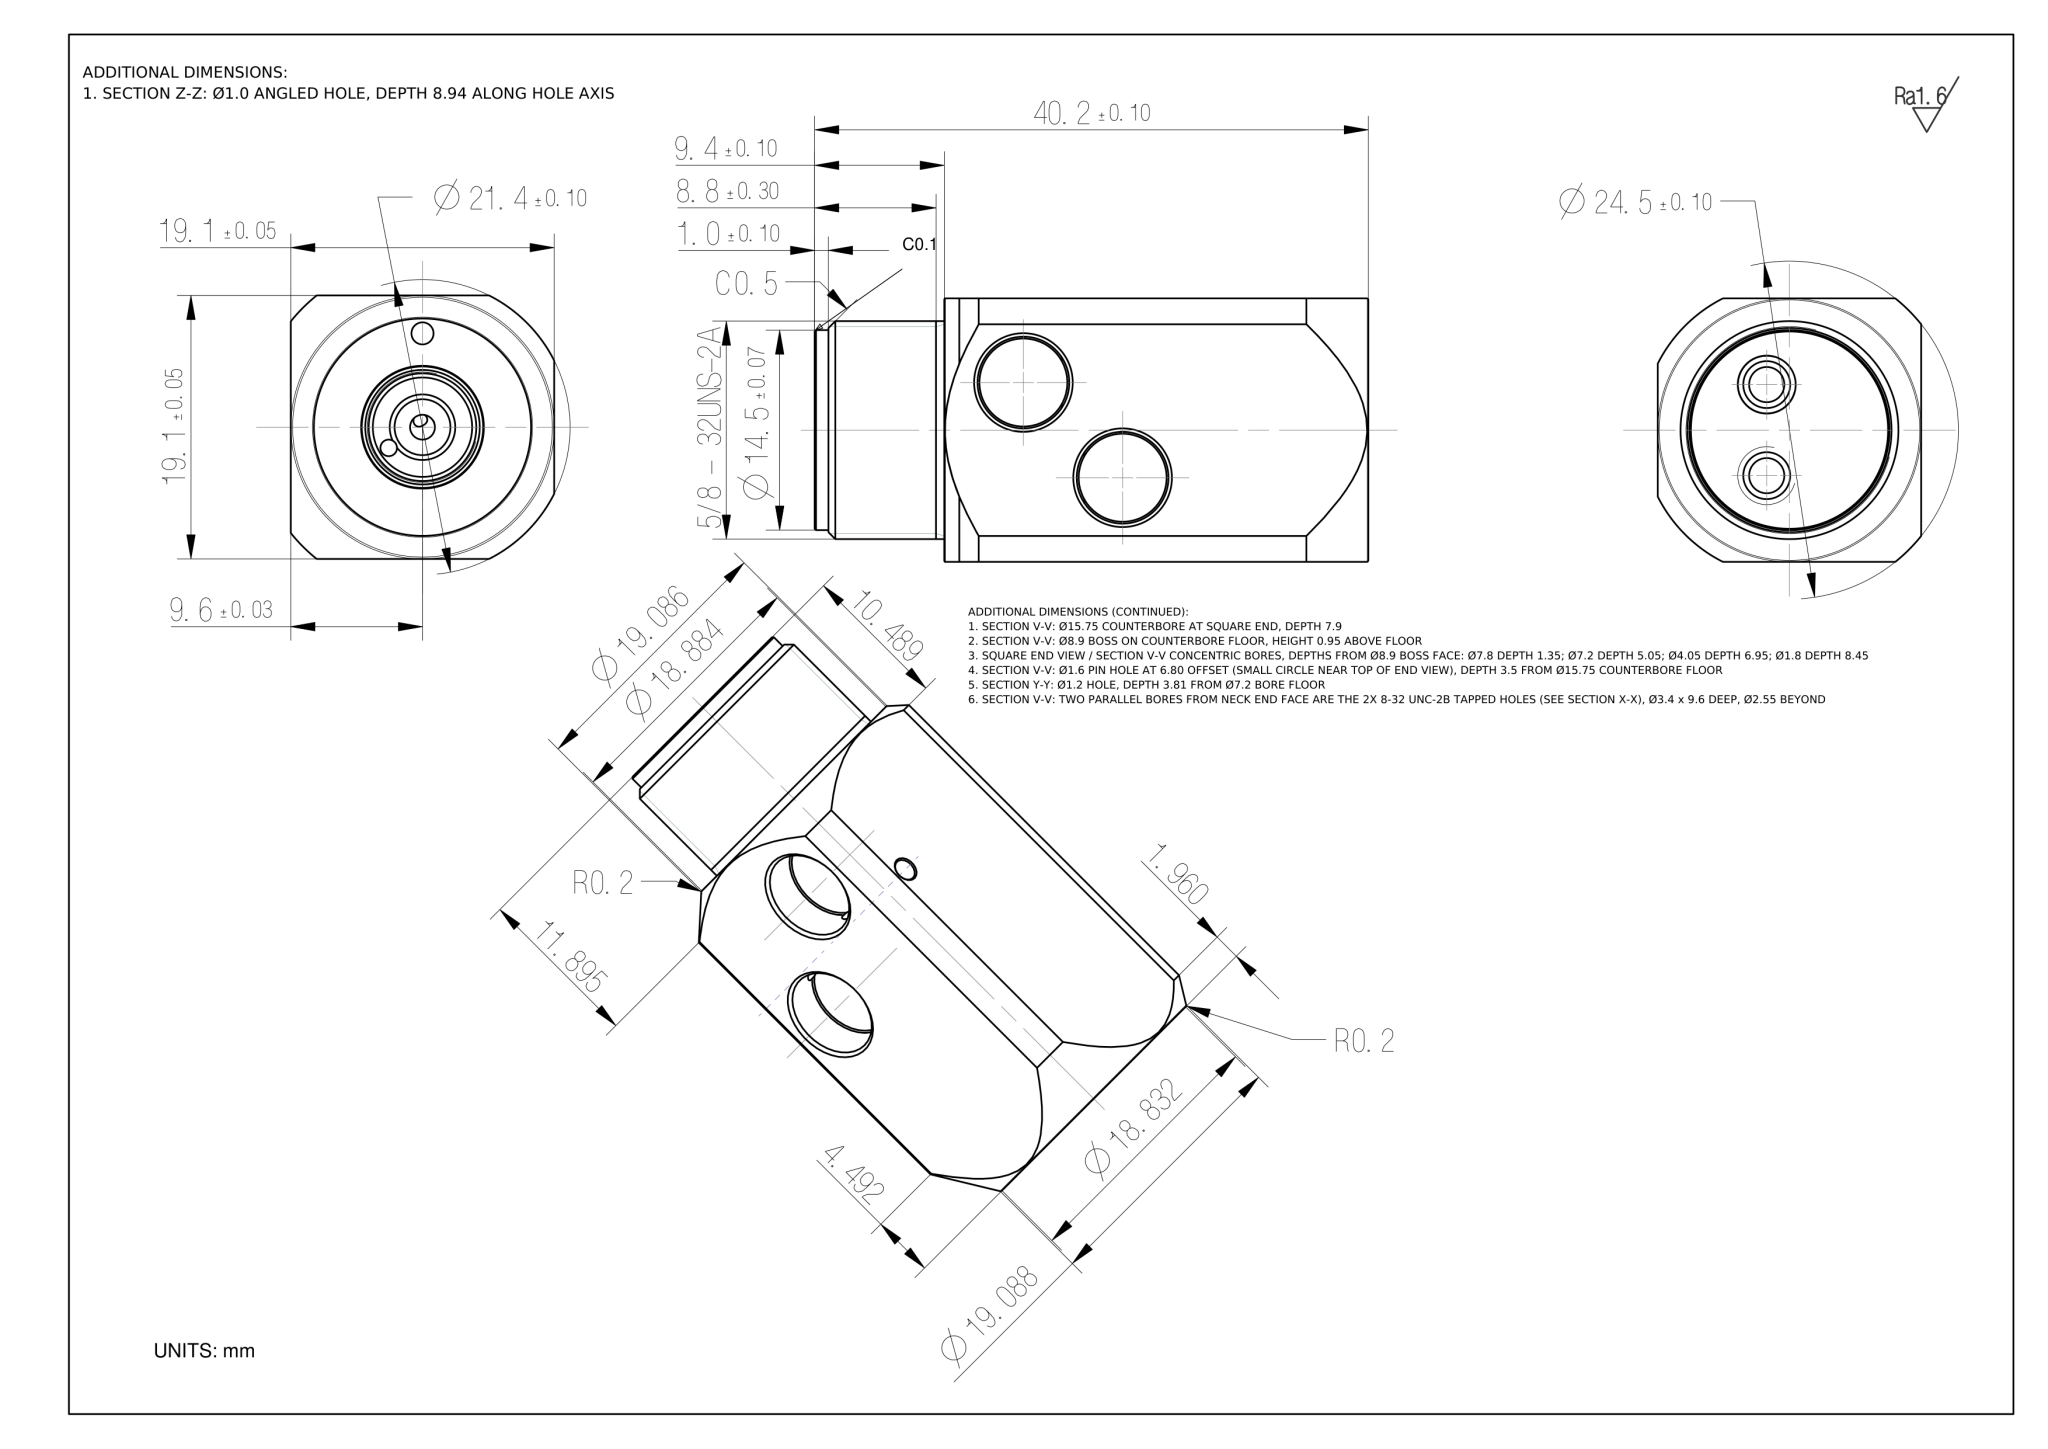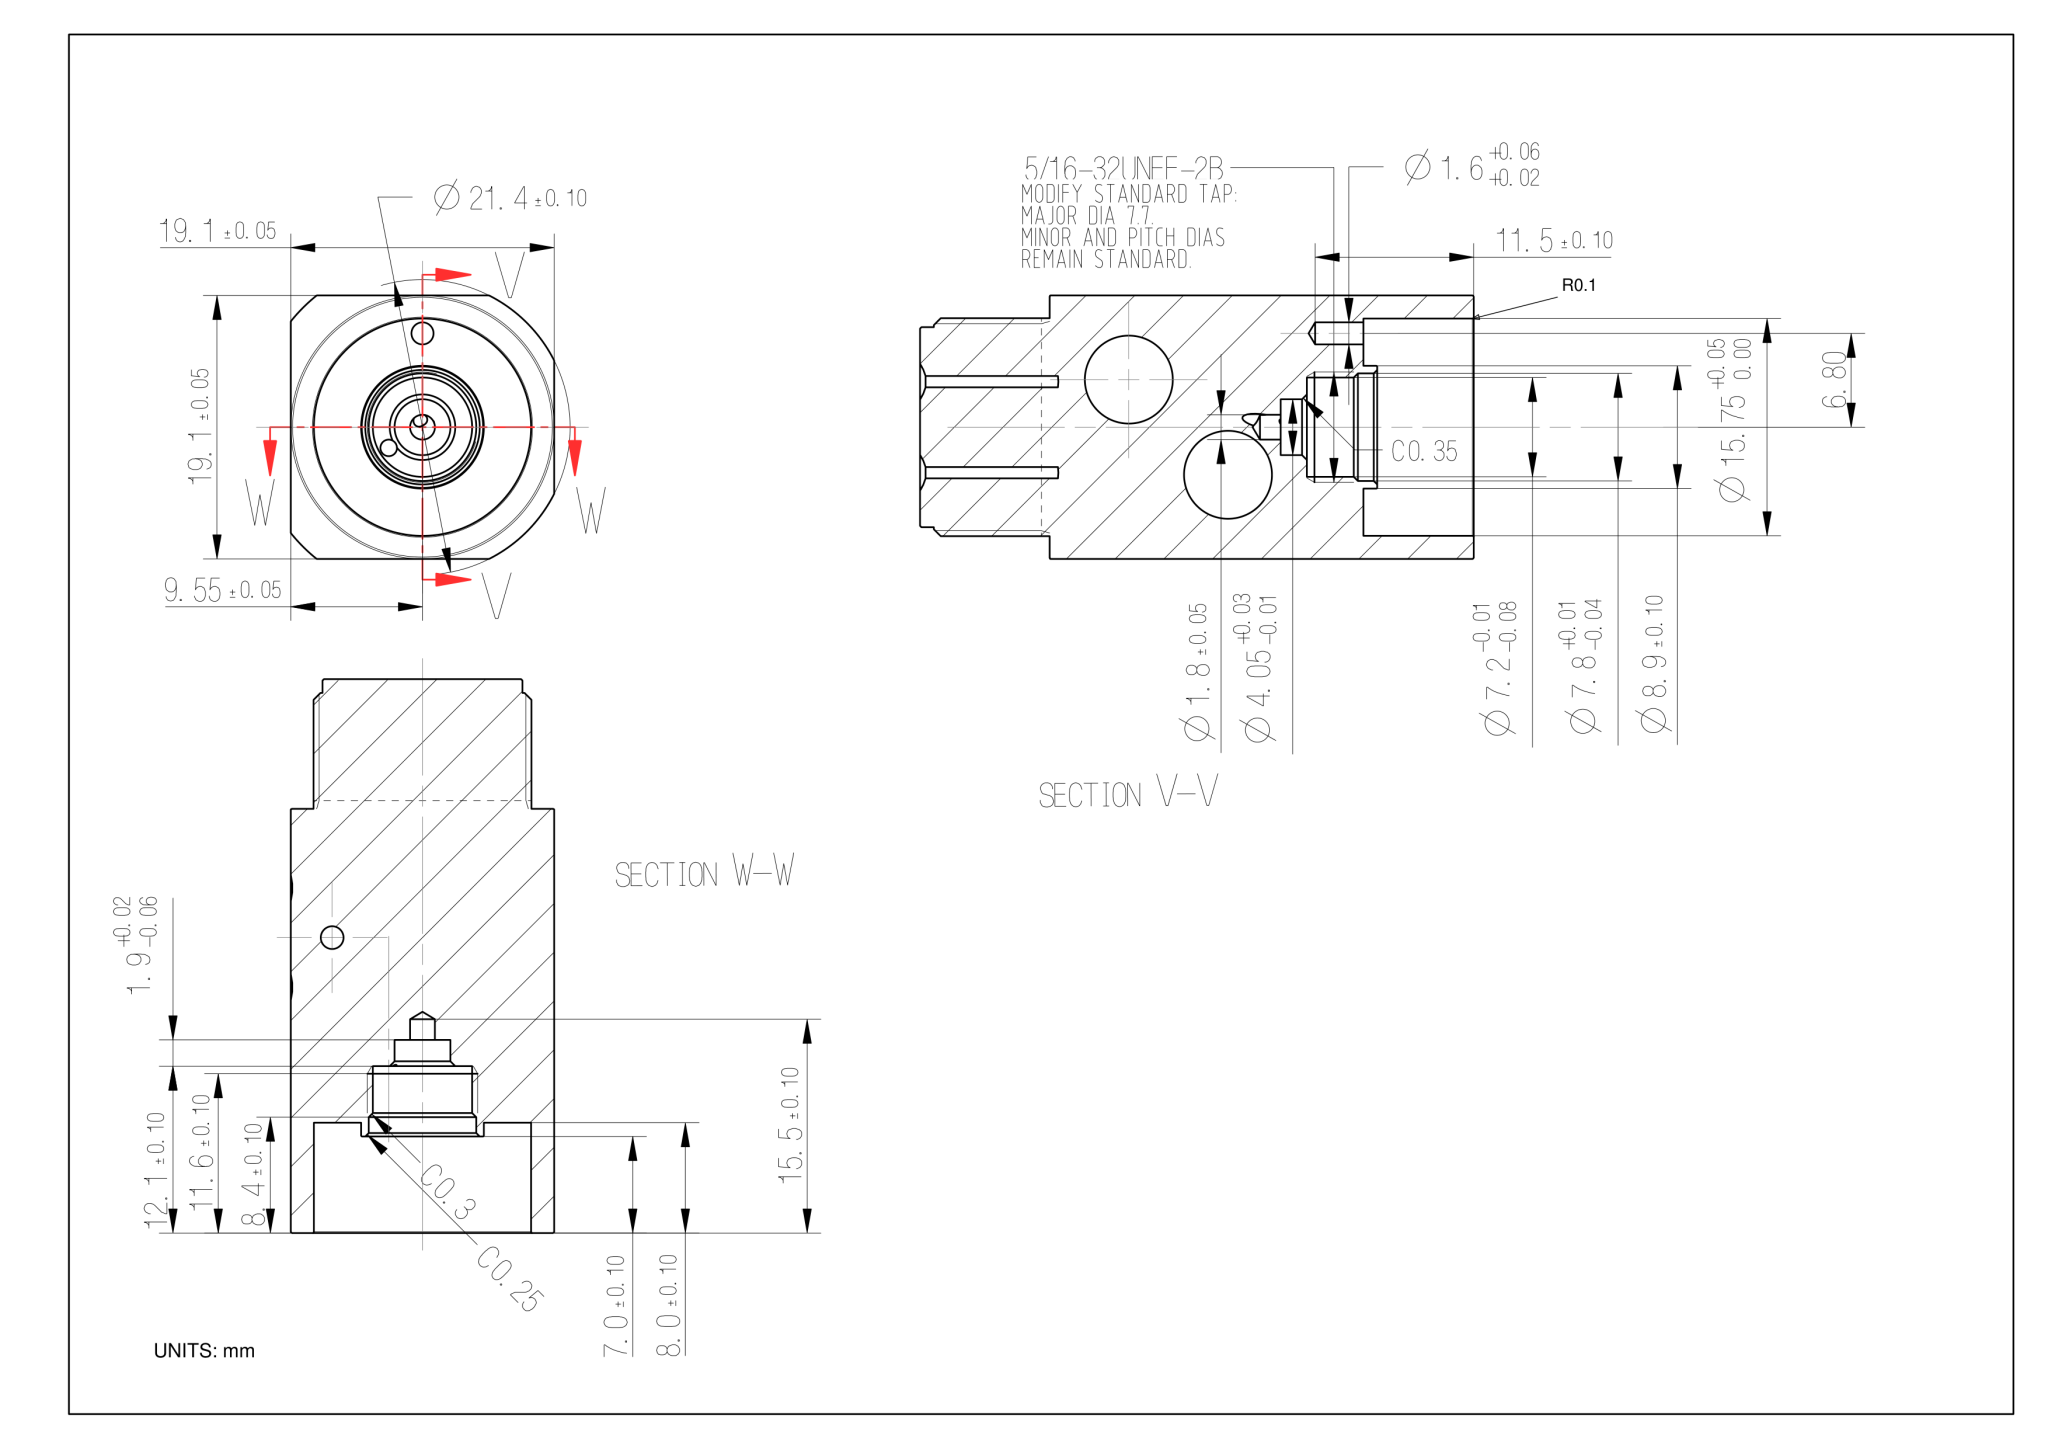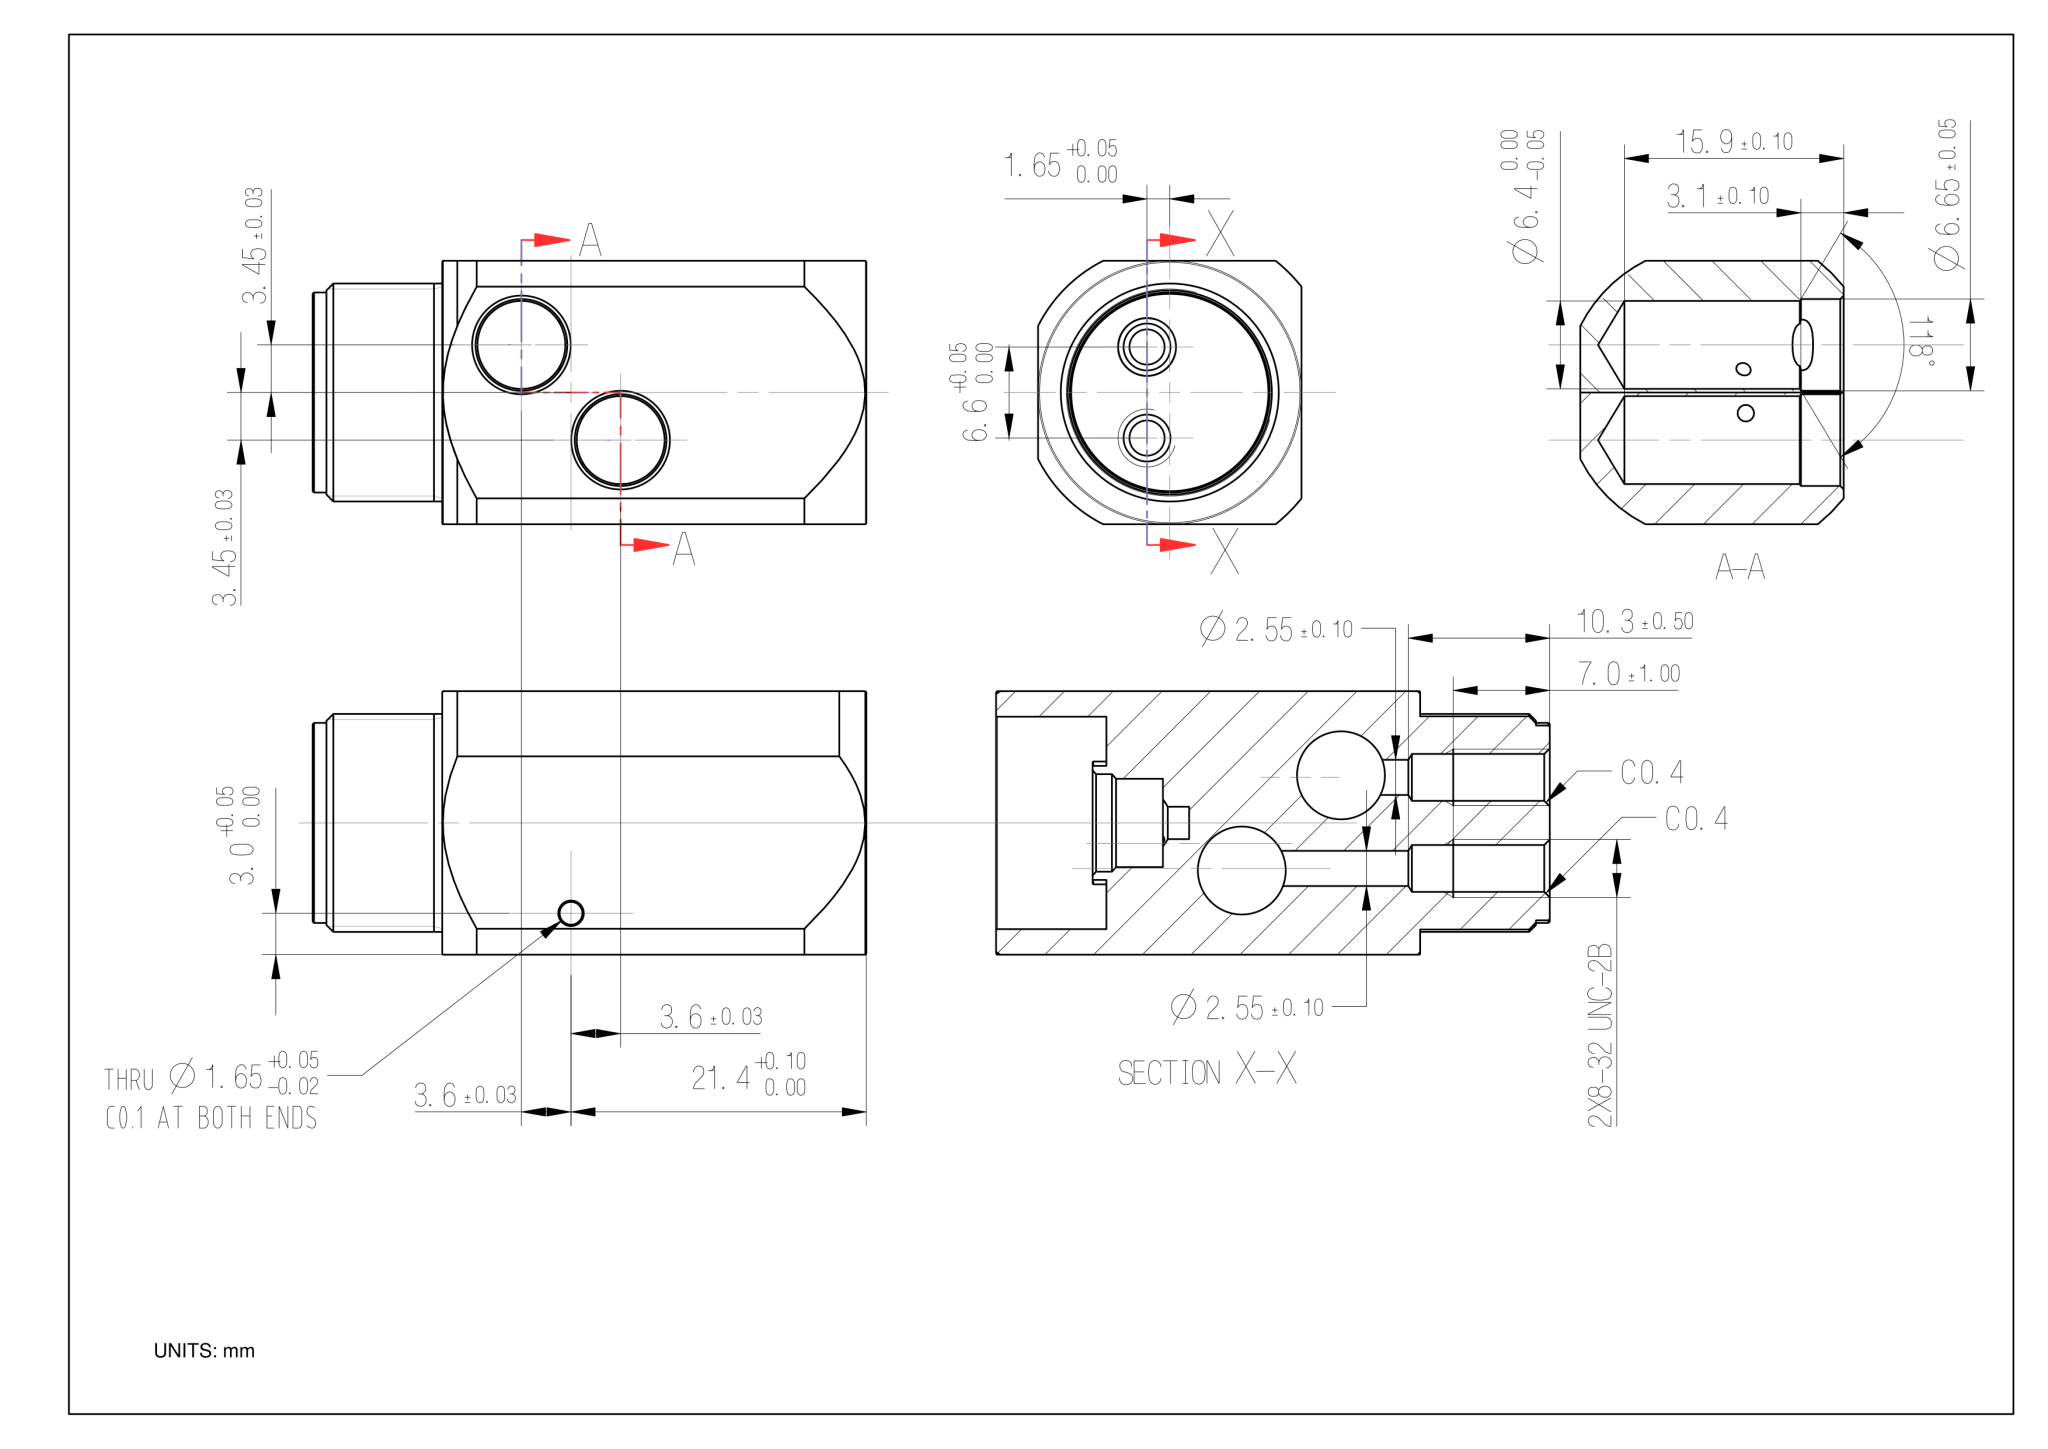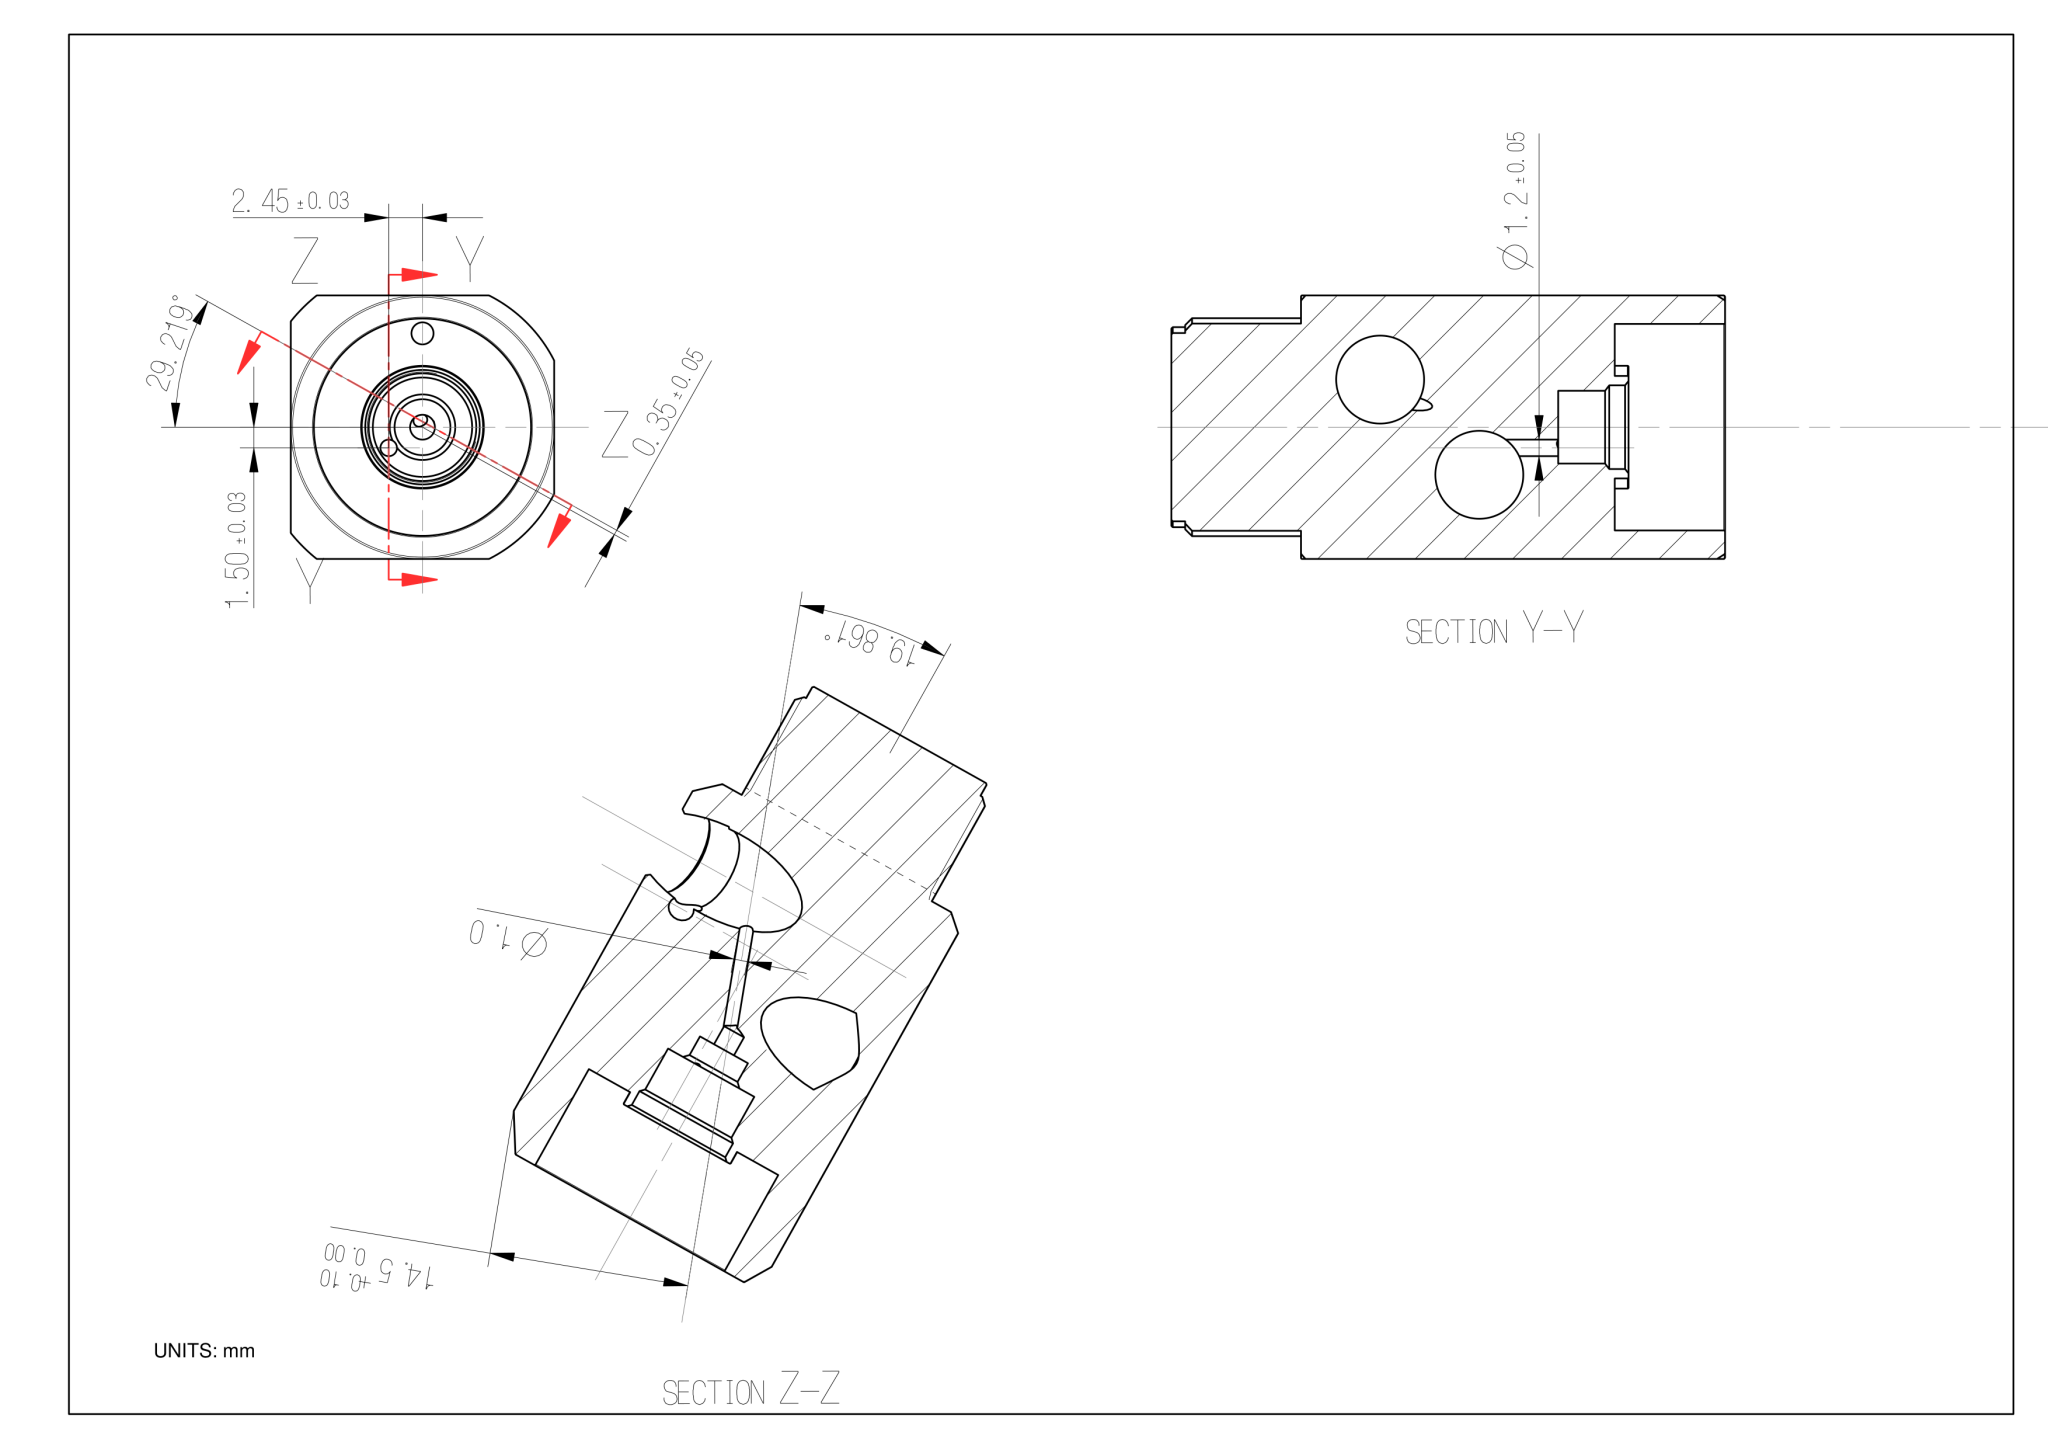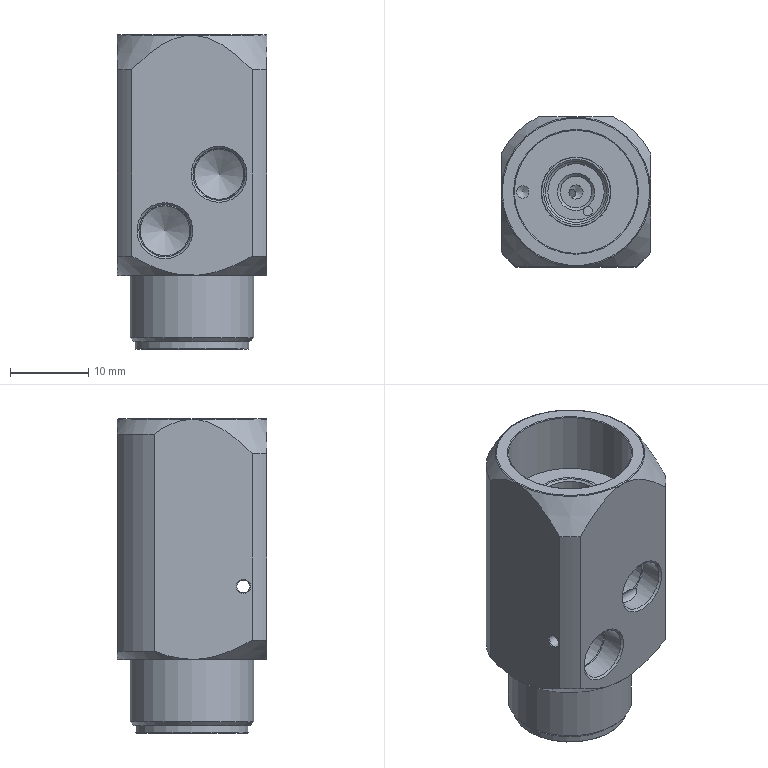Part | NX | mm | 1 solid | 62 faces | box 19.11 x 19.1 x 40.15 mm | volume 9138 mm3 | cylinder 25 | cone 22 | plane 12 | torus 3 | commonest cylinder face diameters 6.65 x2 6.375 x2 21.4 x2 24.5 x2 3.4 x2 2.55 x2 1 x2 15.8 x1